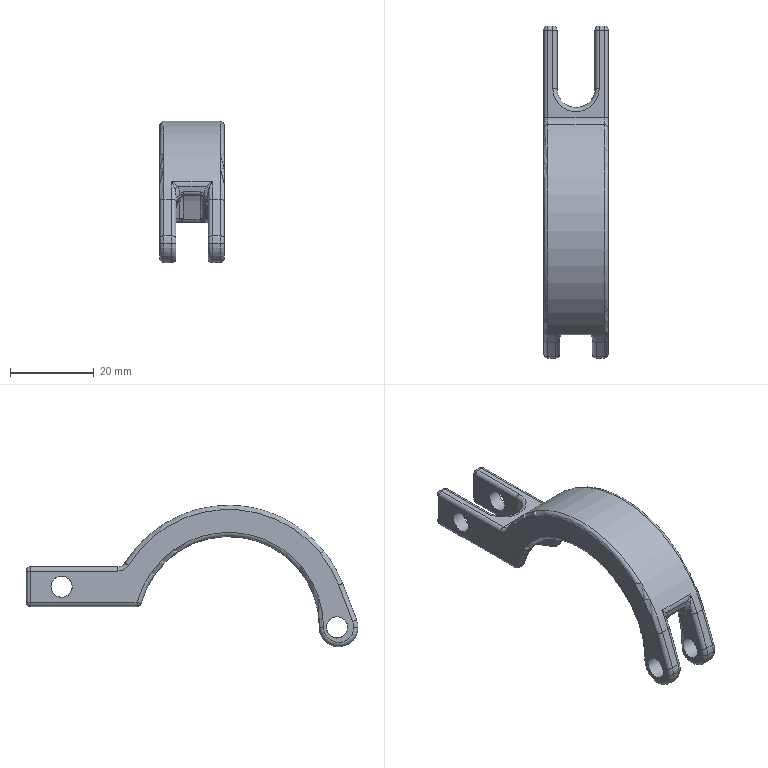Component | NX | UPPER_CLASP | 1 solid | 124 faces | volume 7409 mm3 | cylinder 43 | torus 26 | spline 24 | sphere 16 | plane 13 | cone 2 | commonest cylinder face diameters 2 x28 5.1 x4 10 x2 9.227 x2 43.5 x2 4 x2 58.5 x1 9.1 x1